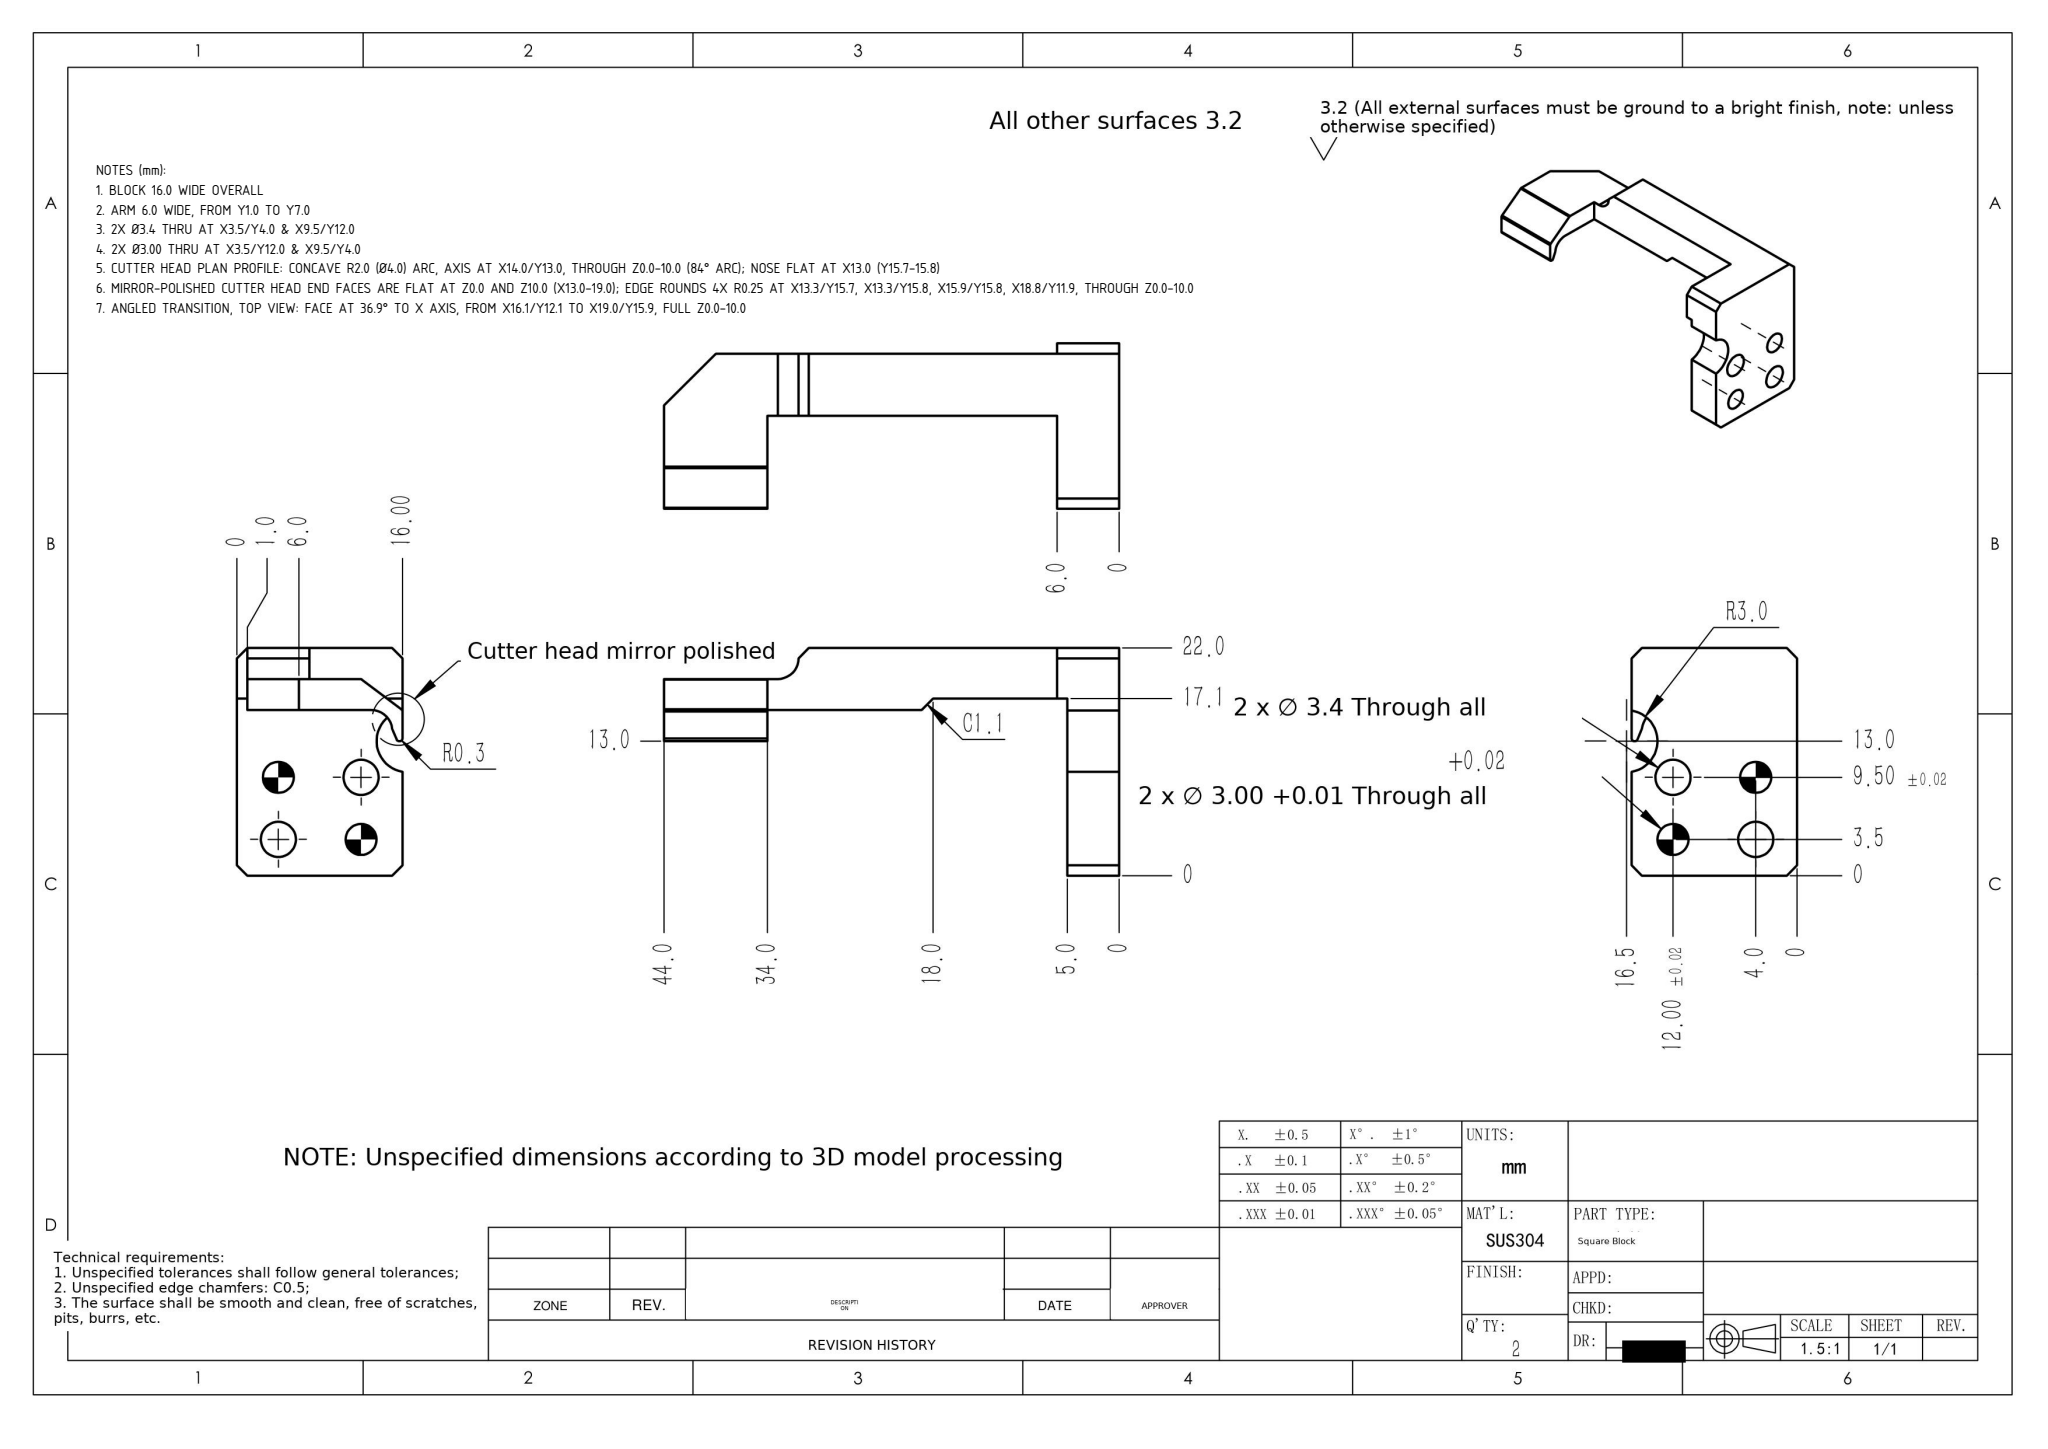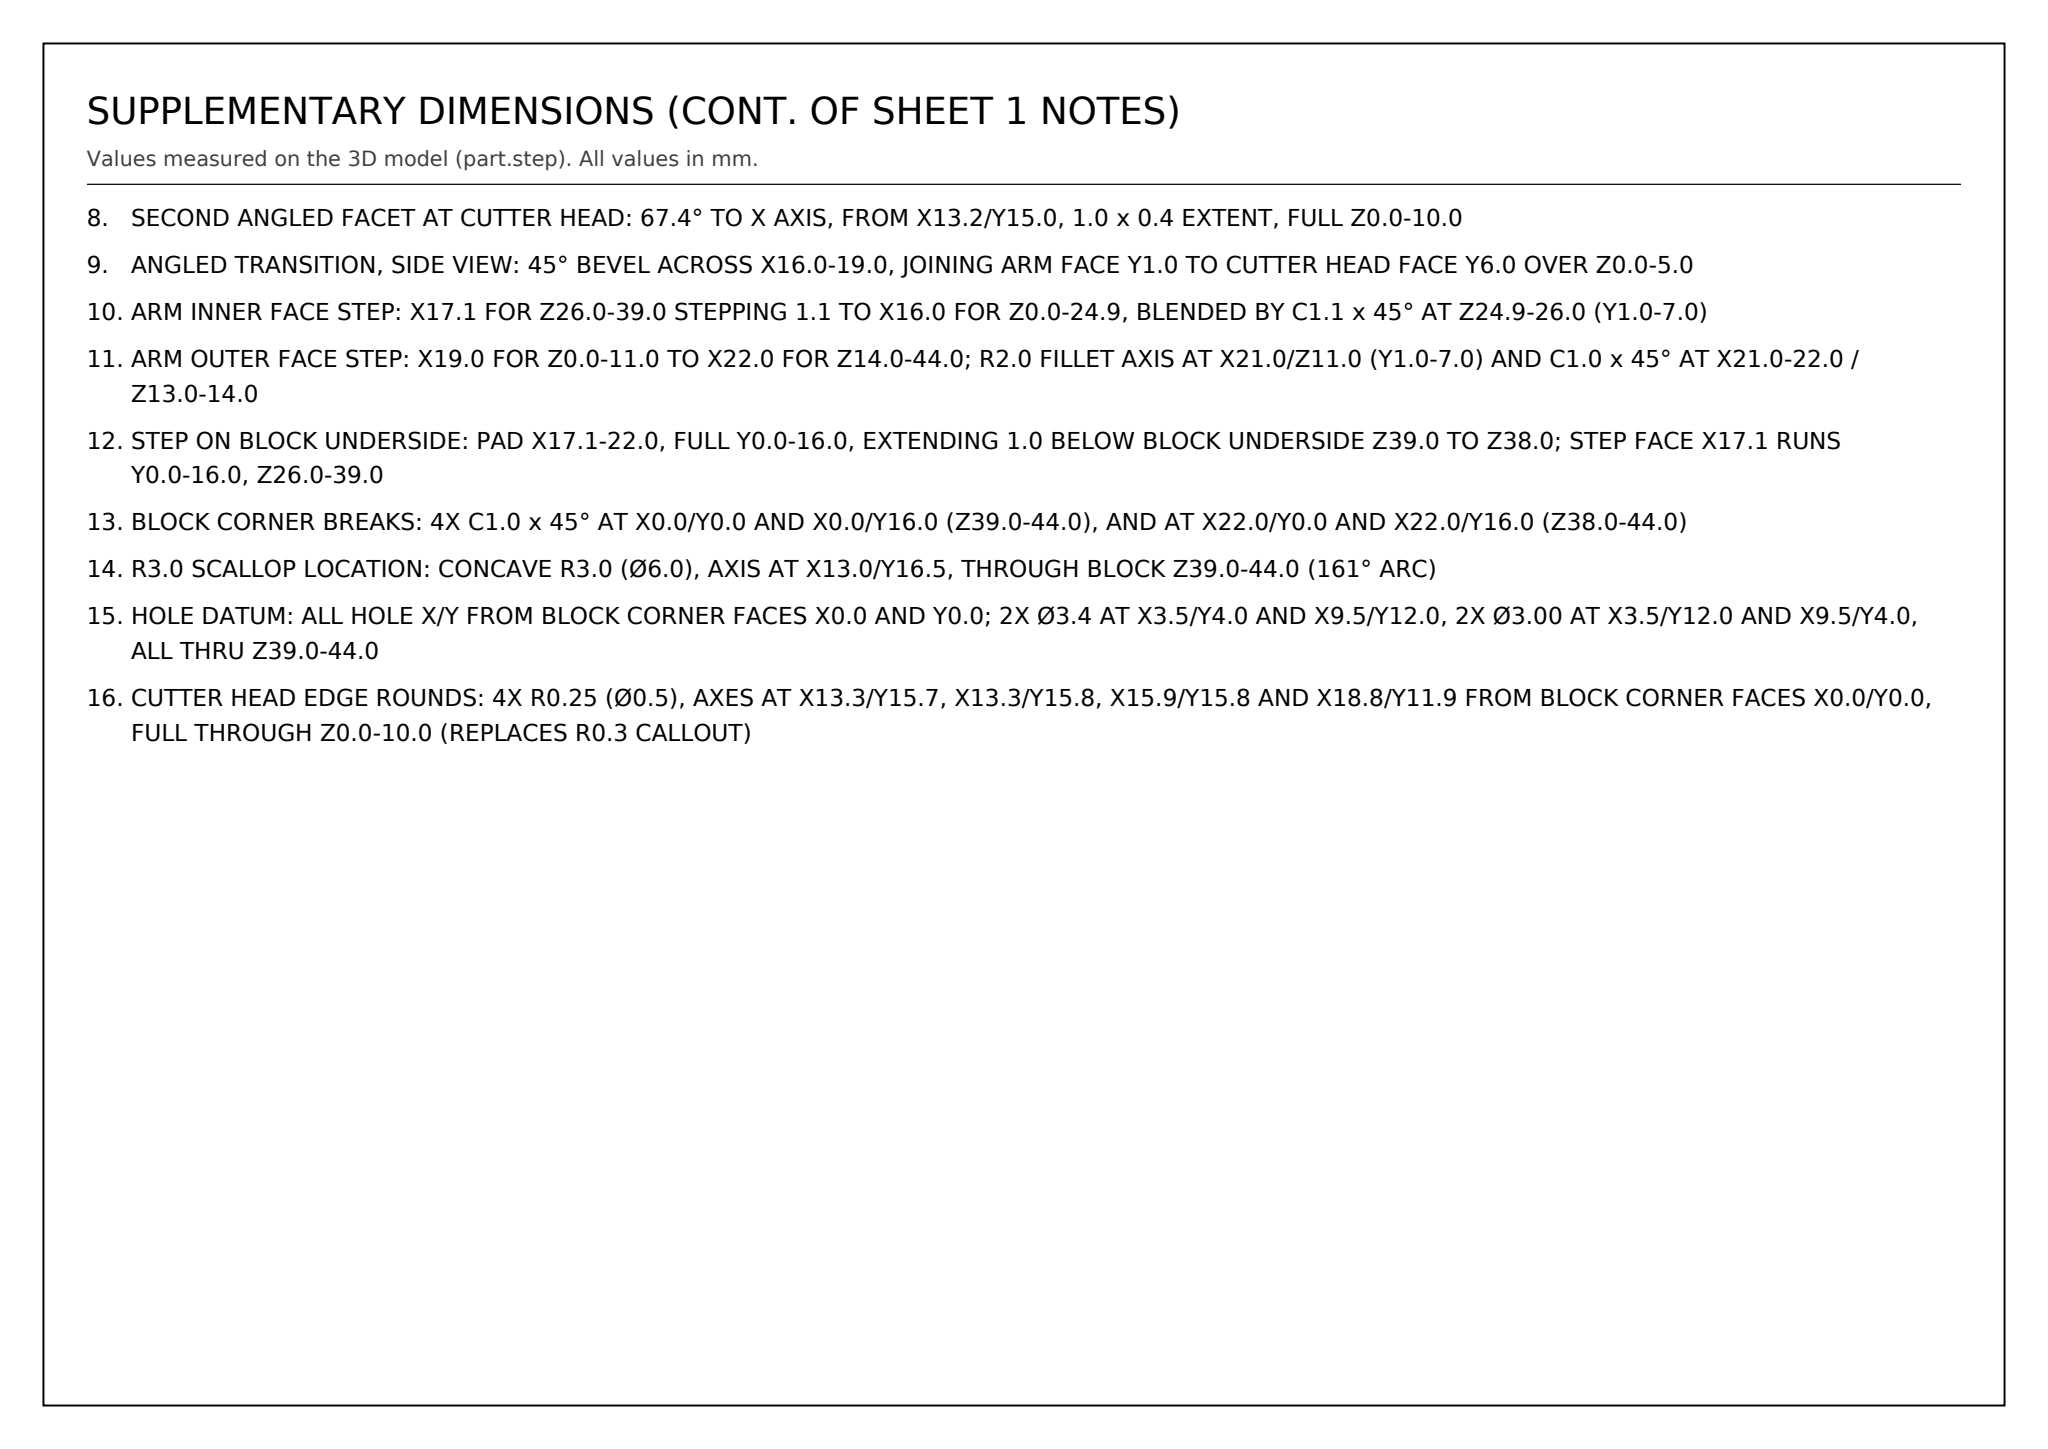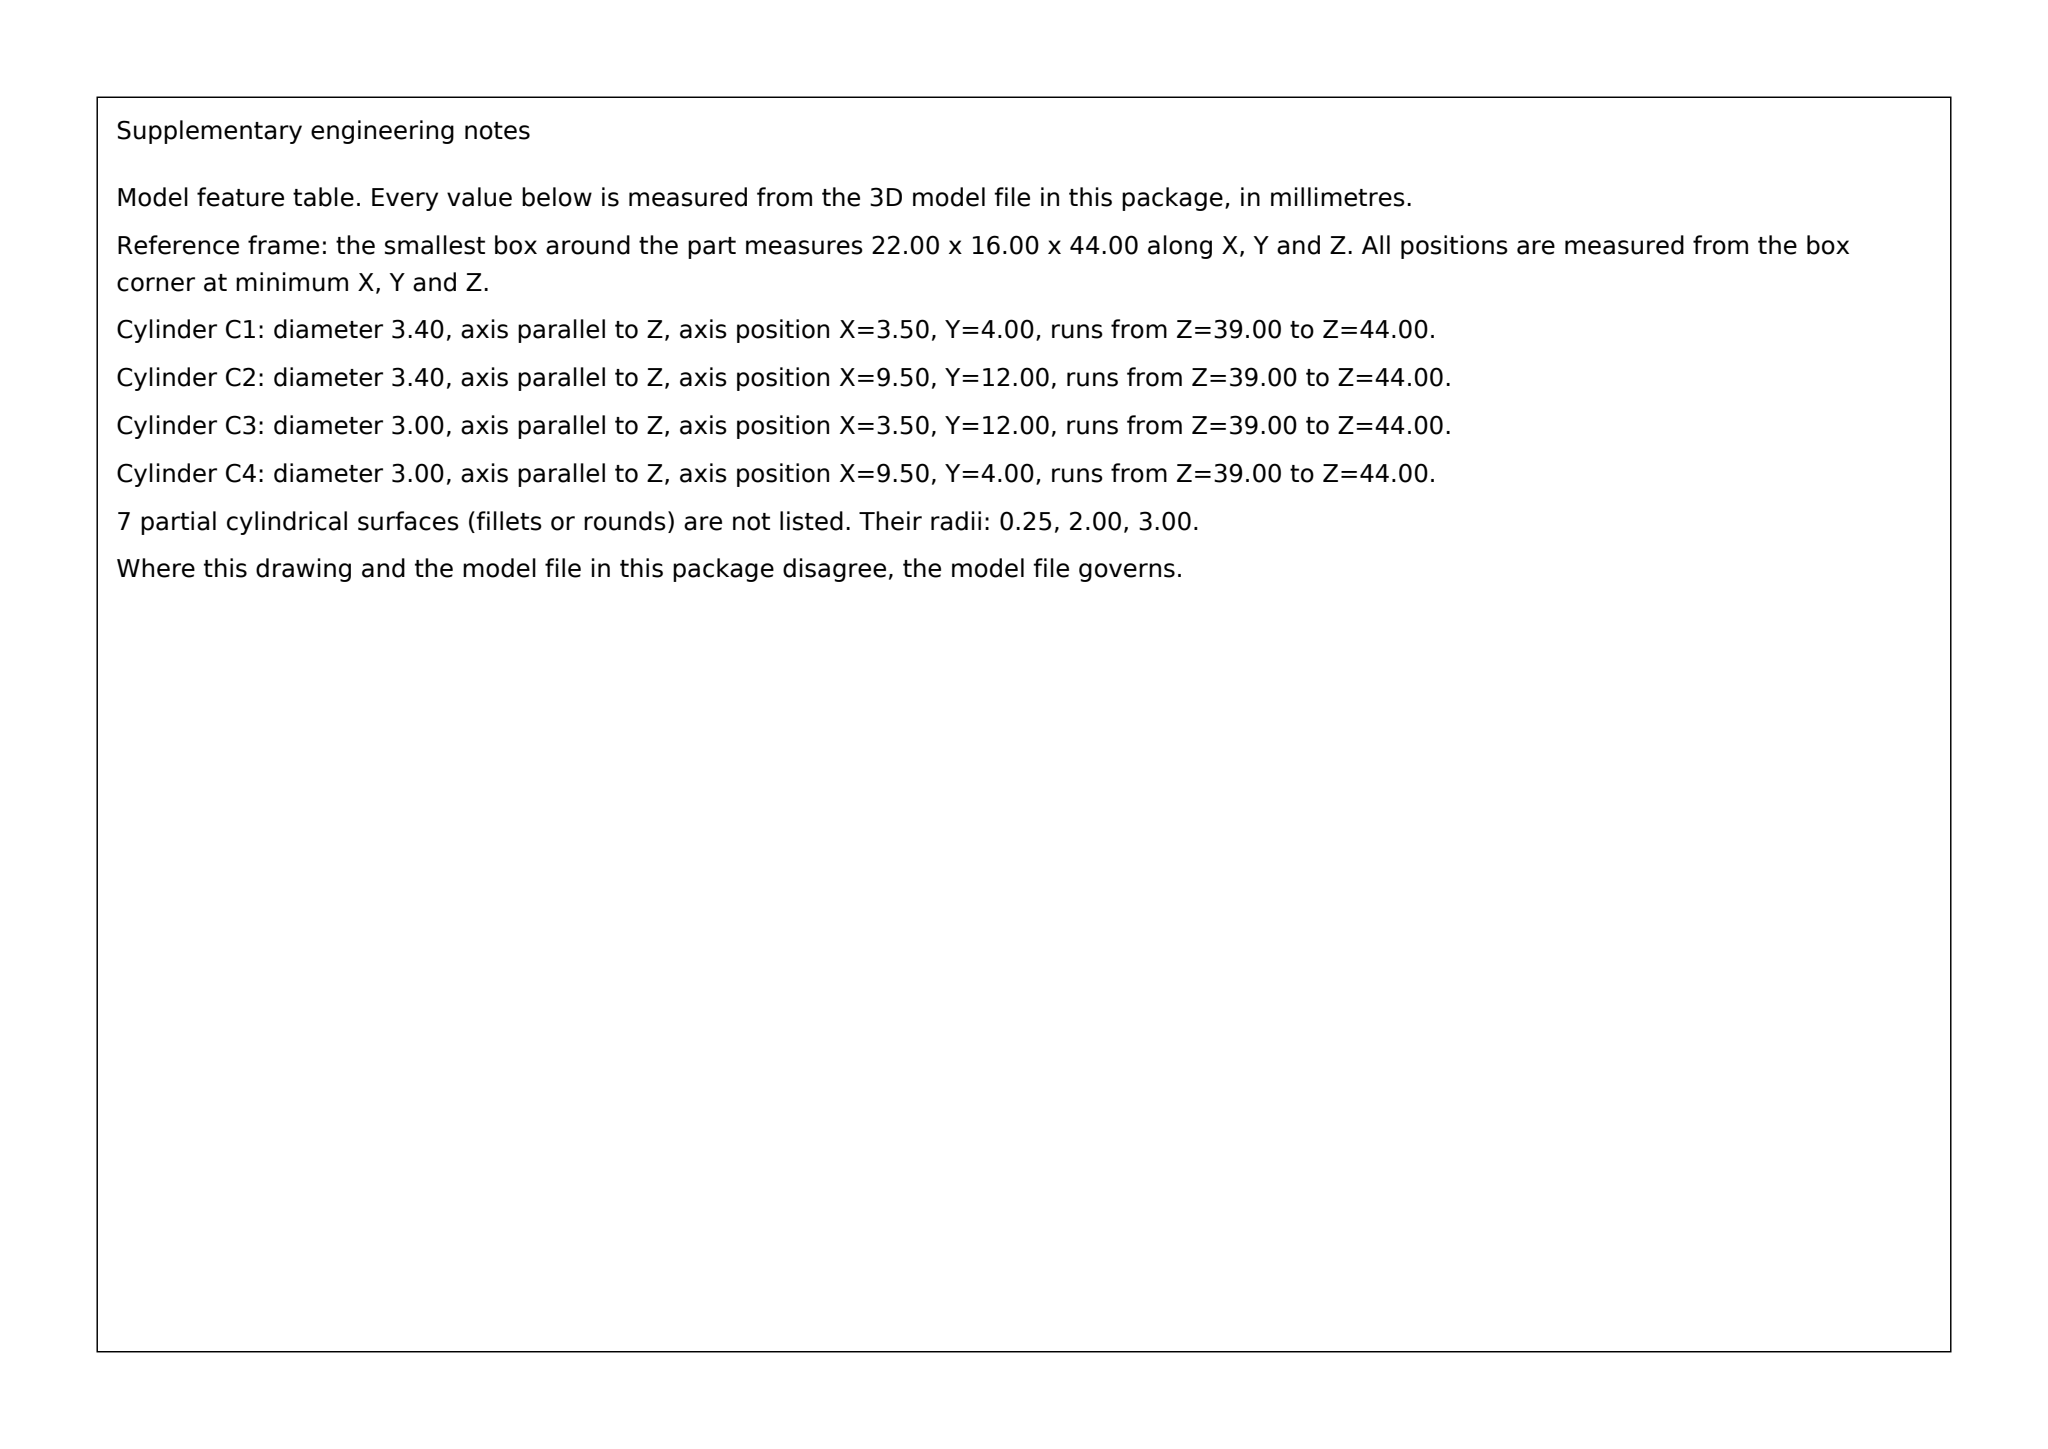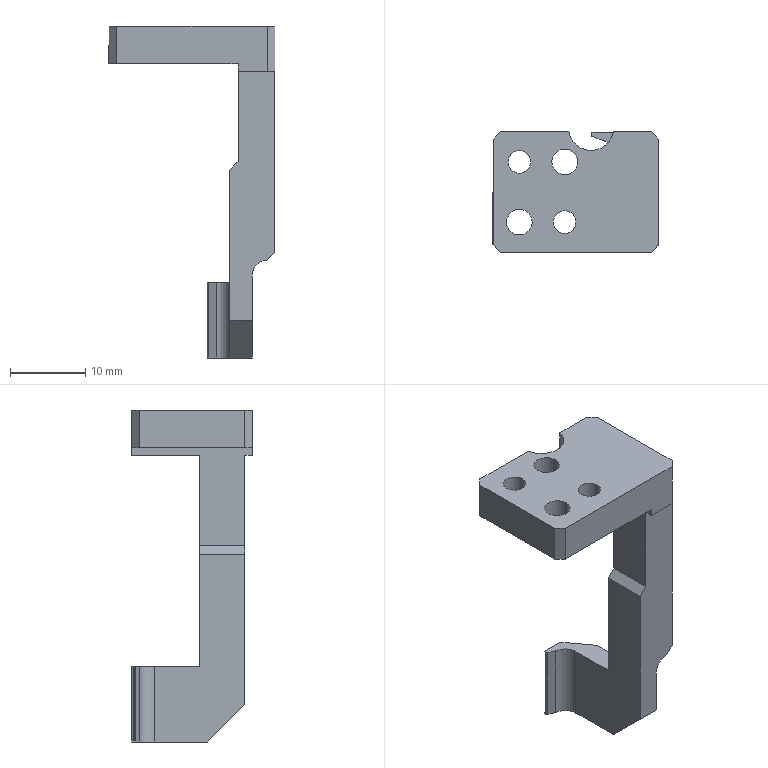Part | SolidWorks | mm | 1 solid | 42 faces | box 22 x 16 x 44 mm | volume 2871 mm3 | plane 27 | cylinder 15 | commonest cylinder face diameters 3.4 x4 3 x4 0.5 x4 4 x2 6 x1
Drawing notes:
BLOCK 16.0 WIDE OVERALL | from the solid: bbox y = 16.0 (end-view 16.5 not supported)
ARM 6.0 WIDE, FROM Y1.0 TO Y7.0 | from the solid: y-planes at 0, 1.0, 7.0, 16.0
2X Ø3.4 THRU AT X3.5/Y4.0 & X9.5/Y12.0 | from the solid: Ø3.4 z-holes at (x3.5,y4.0) & (x9.5,y12.0); end-view horiz ordinate=y, vert=x
2X Ø3.00 THRU AT X3.5/Y12.0 & X9.5/Y4.0 | from the solid: Ø3.0 z-holes at (x3.5,y12.0) & (x9.5,y4.0); end-view horiz ordinate=y, vert=x
CUTTER HEAD PLAN PROFILE: CONCAVE R2.0 (Ø4.0) ARC, AXIS AT X14.0/Y13.0, THROUGH Z0.0-10.0 (84° ARC); NOSE FLAT AT X13.0 (Y15.7-15.8) | from the solid: cylinders: concave arc dia 4.0 axis z at [14.0,13.0] from 0.0 to 10.0, 84 deg; axis_planes x=13.0 extent y[15.7,15.8] z[0,10]
MIRROR-POLISHED CUTTER HEAD END FACES ARE FLAT AT Z0.0 AND Z10.0 (X13.0-19.0); EDGE ROUNDS 4X R0.25 AT X13.3/Y15.7, X13.3/Y15.8, X15.9/Y15.8, X18.8/Y11.9, THROUGH Z0.0-10.0 | from the solid: axis_planes z=0.0 (x13-19,y6-16) and z=10.0 (x13-19,y7-16); cylinders convex arc dia 0.5 axis z at [13.3,15.7],[13.3,15.8],[15.9,15.8],[18.8,11.9] from 0.0 to 10.0
ANGLED TRANSITION, TOP VIEW: FACE AT 36.9° TO X AXIS, FROM X16.1/Y12.1 TO X19.0/Y15.9, FULL Z0.0-10.0 | from the solid: inclined_planes angle_to_xyz_axes [36.9,53.1,90.0], bbox_from [16.1,12.1,0.0], size [2.9,3.8,10.0]
SECOND ANGLED FACET AT CUTTER HEAD: 67.4° TO X AXIS, FROM X13.2/Y15.0, 1.0 x 0.4 EXTENT, FULL Z0.0-10.0 | from the solid: inclined_planes angle_to_xyz_axes [67.4,22.6,90.0], bbox_from [13.2,15.0,0.0], size [1.0,0.4,10.0]
ANGLED TRANSITION, SIDE VIEW: 45° BEVEL ACROSS X16.0-19.0, JOINING ARM FACE Y1.0 TO CUTTER HEAD FACE Y6.0 OVER Z0.0-5.0 | from the solid: inclined_planes angle_to_xyz_axes [90.0,45.0,45.0], bbox_from [16.0,1.0,0.0], size [3.0,5.0,5.0]
ARM INNER FACE STEP: X17.1 FOR Z26.0-39.0 STEPPING 1.1 TO X16.0 FOR Z0.0-24.9, BLENDED BY C1.1 x 45° AT Z24.9-26.0 (Y1.0-7.0) | from the solid: axis_planes x=17.1 (y0-16, z26-39) and x=16.0 (y1-13, z0-24.9); inclined_planes [45.0,90.0,45.0] bbox_from [16.0,1.0,24.9] size [1.1,6.0,1.1]
ARM OUTER FACE STEP: X19.0 FOR Z0.0-11.0 TO X22.0 FOR Z14.0-44.0; R2.0 FILLET AXIS AT X21.0/Z11.0 (Y1.0-7.0) AND C1.0 x 45° AT X21.0-22.0 / Z13.0-14.0 | from the solid: axis_planes x=19.0 (y1-11.9, z0-11) and x=22.0 (y1-15, z14-44); cylinders concave arc dia 4.0 axis y at [21.0,-,11.0] from 1.0 to 7.0, 90 deg; inclined_planes [45.0,90.0,45.0] bbox_from [21.0,1.0,13.0] size [1.0,6.0,1.0]
STEP ON BLOCK UNDERSIDE: PAD X17.1-22.0, FULL Y0.0-16.0, EXTENDING 1.0 BELOW BLOCK UNDERSIDE Z39.0 TO Z38.0; STEP FACE X17.1 RUNS Y0.0-16.0, Z26.0-39.0 | from the solid: axis_planes z=39.0 (x0-17.1, y0-16), z=38.0 (x17.1-22, y0-1 and y7-16), x=17.1 (y0-16, z26-39)
BLOCK CORNER BREAKS: 4X C1.0 x 45° AT X0.0/Y0.0 AND X0.0/Y16.0 (Z39.0-44.0), AND AT X22.0/Y0.0 AND X22.0/Y16.0 (Z38.0-44.0) | from the solid: inclined_planes [45,45,90] bbox_from [0,0,39] size [1,1,5]; [0,15,39] size [1,1,5]; [21,0,38] size [1,1,6]; [21,15,38] size [1,1,6]
R3.0 SCALLOP LOCATION: CONCAVE R3.0 (Ø6.0), AXIS AT X13.0/Y16.5, THROUGH BLOCK Z39.0-44.0 (161° ARC) | from the solid: cylinders concave arc dia 6.0 axis z at [13.0,16.5] from 39.0 to 44.0, 161 deg
HOLE DATUM: ALL HOLE X/Y FROM BLOCK CORNER FACES X0.0 AND Y0.0; 2X Ø3.4 AT X3.5/Y4.0 AND X9.5/Y12.0, 2X Ø3.00 AT X3.5/Y12.0 AND X9.5/Y4.0, ALL THRU Z39.0-44.0 | from the solid: cylinders hole/bore dia 3.4 axis z at [3.5,4.0] and [9.5,12.0]; dia 3.0 axis z at [3.5,12.0] and [9.5,4.0]; all from 39.0 to 44.0
CUTTER HEAD EDGE ROUNDS: 4X R0.25 (Ø0.5), AXES AT X13.3/Y15.7, X13.3/Y15.8, X15.9/Y15.8 AND X18.8/Y11.9 FROM BLOCK CORNER FACES X0.0/Y0.0, FULL THROUGH Z0.0-10.0 (REPLACES R0.3 CALLOUT) | from the solid: cylinders: 4X convex arc (round/outer radius) dia 0.5, axis z at [13.3,15.7], [13.3,15.8], [15.9,15.8], [18.8,11.9], from z0.0 to z10.0